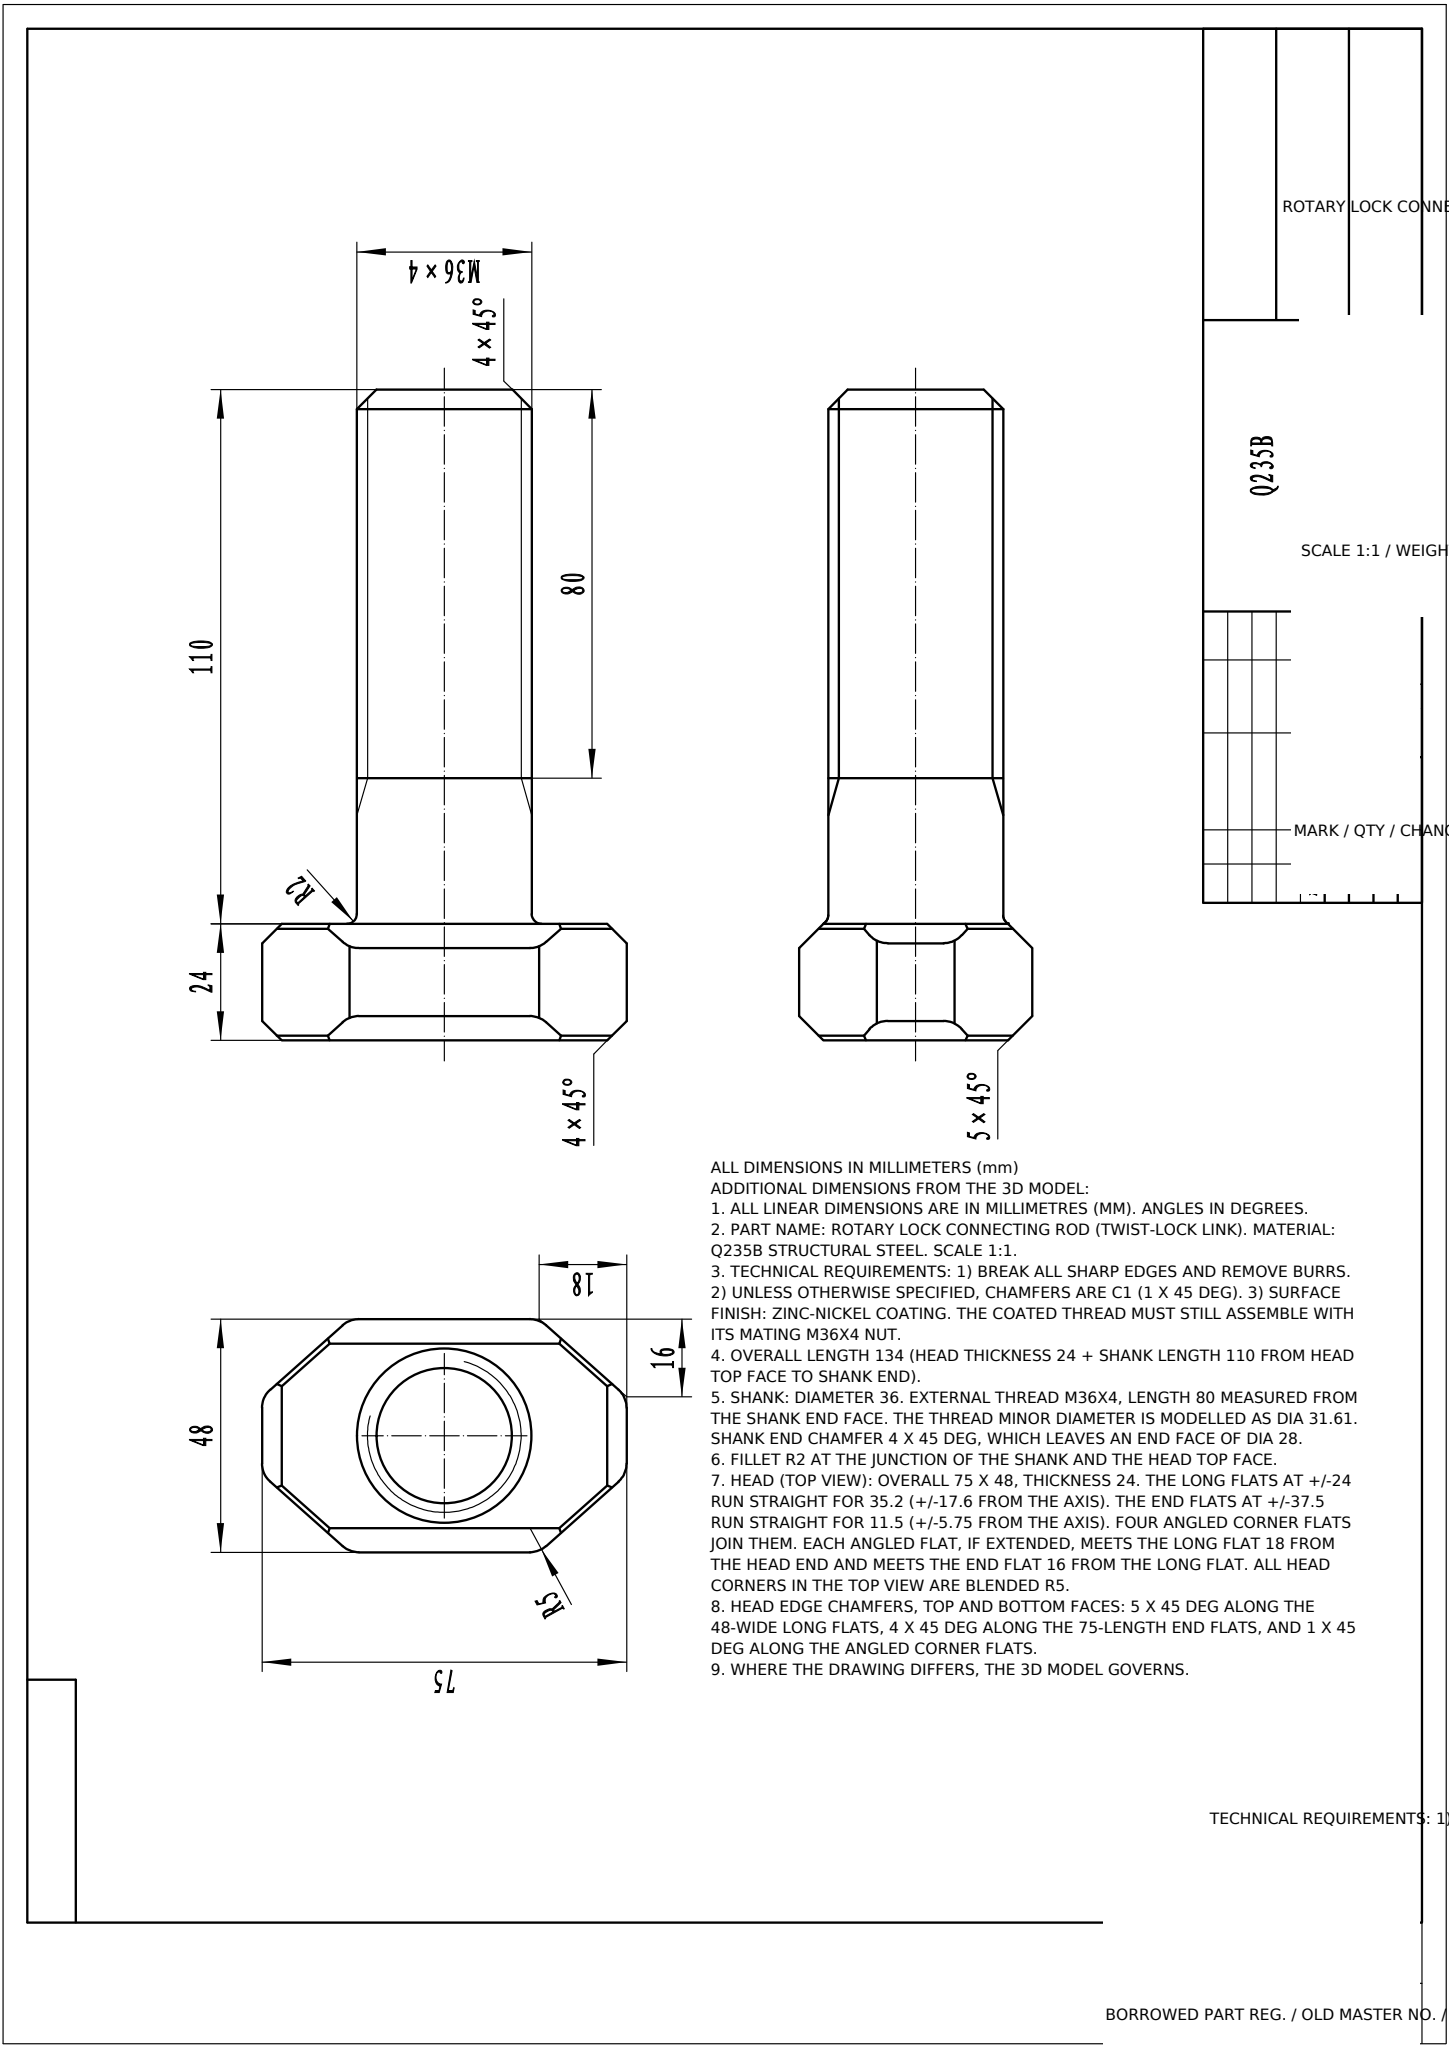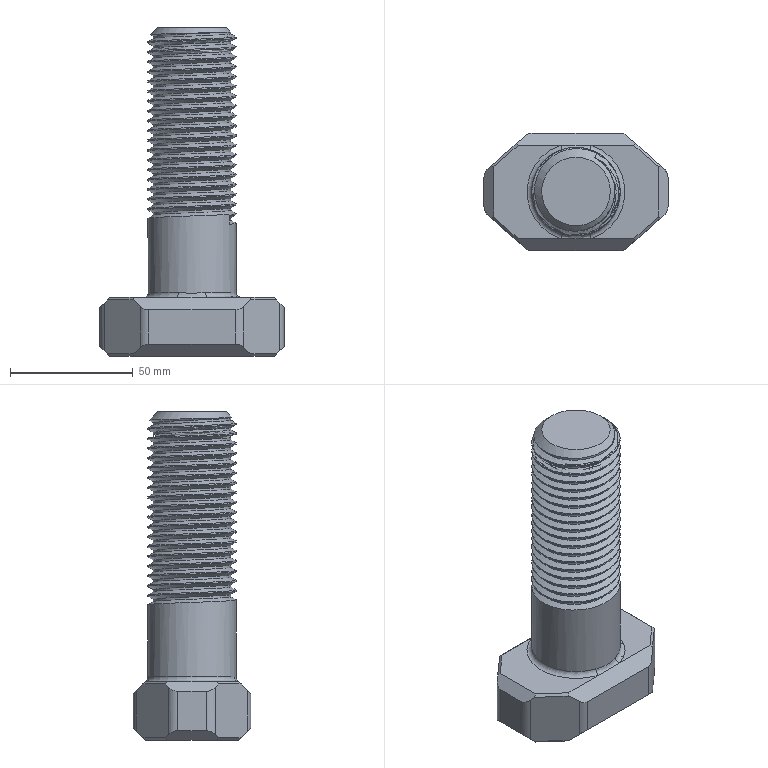Part | NX | mm | 1 solid | 65 faces | box 75 x 48 x 134 mm | volume 170587 mm3 | plane 29 | cylinder 28 | spline 4 | cone 2 | torus 2 | commonest cylinder face diameters 36 x19 10 x8 31.61 x1